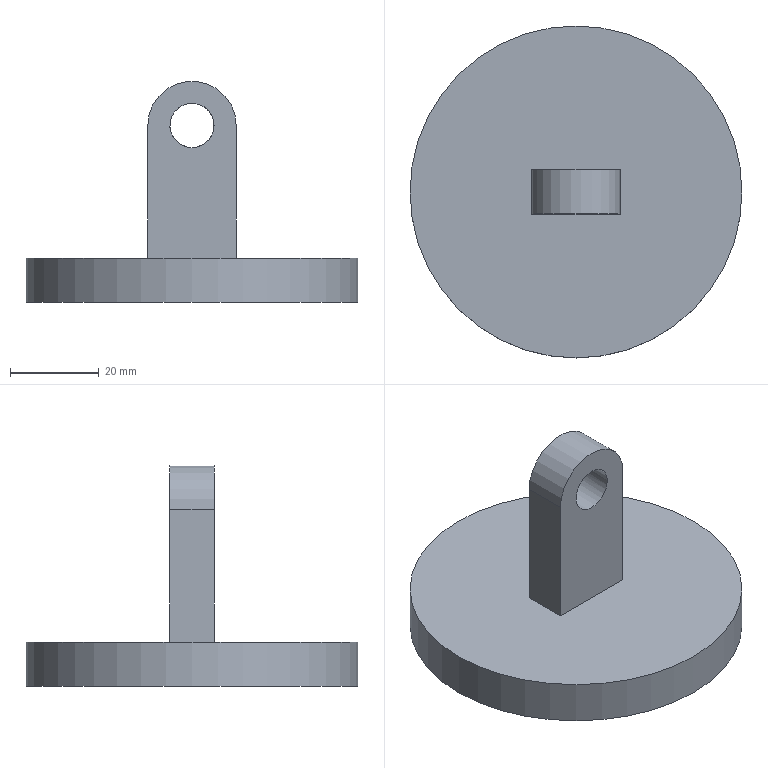Component | NX | CIRCLE_PISTON | 1 solid | 9 faces | box 75 x 75 x 50 mm | volume 50964 mm3 | plane 6 | cylinder 3 | commonest cylinder face diameters 75 x1 20 x1 10 x1
STEP:
#1=CARTESIAN_POINT('',(0.,0.,0.));
#2=DIRECTION('',(0.,0.,1.));
#3=DIRECTION('',(1.,0.,0.));
#4=AXIS2_PLACEMENT_3D('',#1,#2,#3);
#5=CARTESIAN_POINT('',(-162.5,20.,60.412));
#6=VERTEX_POINT('',#5);
#7=CARTESIAN_POINT('',(-200.,20.,60.412));
#8=DIRECTION('',(0.,0.,1.));
#9=DIRECTION('',(1.,0.,0.));
#10=AXIS2_PLACEMENT_3D('',#7,#8,#9);
#11=CIRCLE('',#10,37.5);
#12=CARTESIAN_POINT('',(-200.,20.,60.412));
#13=DIRECTION('',(0.,0.,1.));
#14=DIRECTION('',(1.,0.,0.));
#15=AXIS2_PLACEMENT_3D('',#12,#13,#14);
#16=PLANE('',#15);
#17=CARTESIAN_POINT('',(0.,0.));
#18=DIRECTION('',(1.,0.));
#19=AXIS2_PLACEMENT_2D('',#17,#18);
#20=CIRCLE('',#19,37.5);
#21=(GEOMETRIC_REPRESENTATION_CONTEXT(2)PARAMETRIC_REPRESENTATION_CONTEXT()REPRESENTATION_CONTEXT('',''));
#22=DEFINITIONAL_REPRESENTATION('',(#20),#21);
#23=PCURVE('',#16,#22);
#24=CARTESIAN_POINT('',(-200.,20.,60.412));
#25=DIRECTION('',(0.,0.,-1.));
#26=DIRECTION('',(-1.,0.,0.));
#27=AXIS2_PLACEMENT_3D('',#24,#25,#26);
#28=CYLINDRICAL_SURFACE('',#27,37.5);
#29=CARTESIAN_POINT('',(9.425,0.));
#30=DIRECTION('',(-1.,0.));
#31=VECTOR('',#30,1.);
#32=LINE('',#29,#31);
#33=(GEOMETRIC_REPRESENTATION_CONTEXT(2)PARAMETRIC_REPRESENTATION_CONTEXT()REPRESENTATION_CONTEXT('',''));
#34=DEFINITIONAL_REPRESENTATION('',(#32),#33);
#35=PCURVE('',#28,#34);
#36=SURFACE_CURVE('',#11,(#23,#35),.PCURVE_S1.);
#37=EDGE_CURVE('',#6,#6,#36,.T.);
#38=ORIENTED_EDGE('',*,*,#37,.T.);
#39=EDGE_LOOP('',(#38));
#40=FACE_BOUND('',#39,.T.);
#41=CARTESIAN_POINT('',(-210.,15.,60.412));
#42=VERTEX_POINT('',#41);
#43=CARTESIAN_POINT('',(-210.,25.,60.412));
#44=VERTEX_POINT('',#43);
#45=CARTESIAN_POINT('',(-210.,15.,60.412));
#46=DIRECTION('',(0.,1.,0.));
#47=VECTOR('',#46,1.);
#48=LINE('',#45,#47);
#49=CARTESIAN_POINT('',(-10.,-5.));
#50=DIRECTION('',(0.,1.));
#51=VECTOR('',#50,1.);
#52=LINE('',#49,#51);
#53=(GEOMETRIC_REPRESENTATION_CONTEXT(2)PARAMETRIC_REPRESENTATION_CONTEXT()REPRESENTATION_CONTEXT('',''));
#54=DEFINITIONAL_REPRESENTATION('',(#52),#53);
#55=PCURVE('',#16,#54);
#56=CARTESIAN_POINT('',(-210.,15.,90.412));
#57=DIRECTION('',(1.,0.,0.));
#58=DIRECTION('',(0.,0.,-1.));
#59=AXIS2_PLACEMENT_3D('',#56,#57,#58);
#60=PLANE('',#59);
#61=CARTESIAN_POINT('',(30.,0.));
#62=DIRECTION('',(0.,1.));
#63=VECTOR('',#62,1.);
#64=LINE('',#61,#63);
#65=(GEOMETRIC_REPRESENTATION_CONTEXT(2)PARAMETRIC_REPRESENTATION_CONTEXT()REPRESENTATION_CONTEXT('',''));
#66=DEFINITIONAL_REPRESENTATION('',(#64),#65);
#67=PCURVE('',#60,#66);
#68=SURFACE_CURVE('',#48,(#55,#67),.PCURVE_S1.);
#69=EDGE_CURVE('',#42,#44,#68,.T.);
#70=ORIENTED_EDGE('',*,*,#69,.T.);
#71=CARTESIAN_POINT('',(-190.,25.,60.412));
#72=VERTEX_POINT('',#71);
#73=CARTESIAN_POINT('',(-210.,25.,60.412));
#74=DIRECTION('',(1.,0.,-0.));
#75=VECTOR('',#74,1.);
#76=LINE('',#73,#75);
#77=CARTESIAN_POINT('',(-10.,5.));
#78=DIRECTION('',(1.,0.));
#79=VECTOR('',#78,1.);
#80=LINE('',#77,#79);
#81=(GEOMETRIC_REPRESENTATION_CONTEXT(2)PARAMETRIC_REPRESENTATION_CONTEXT()REPRESENTATION_CONTEXT('',''));
#82=DEFINITIONAL_REPRESENTATION('',(#80),#81);
#83=PCURVE('',#16,#82);
#84=CARTESIAN_POINT('',(-200.,25.,90.412));
#85=DIRECTION('',(0.,-1.,0.));
#86=DIRECTION('',(0.,0.,-1.));
#87=AXIS2_PLACEMENT_3D('',#84,#85,#86);
#88=PLANE('',#87);
#89=CARTESIAN_POINT('',(30.,-10.));
#90=DIRECTION('',(0.,1.));
#91=VECTOR('',#90,1.);
#92=LINE('',#89,#91);
#93=(GEOMETRIC_REPRESENTATION_CONTEXT(2)PARAMETRIC_REPRESENTATION_CONTEXT()REPRESENTATION_CONTEXT('',''));
#94=DEFINITIONAL_REPRESENTATION('',(#92),#93);
#95=PCURVE('',#88,#94);
#96=SURFACE_CURVE('',#76,(#83,#95),.PCURVE_S1.);
#97=EDGE_CURVE('',#44,#72,#96,.T.);
#98=ORIENTED_EDGE('',*,*,#97,.T.);
#99=CARTESIAN_POINT('',(-190.,15.,60.412));
#100=VERTEX_POINT('',#99);
#101=CARTESIAN_POINT('',(-190.,15.,60.412));
#102=DIRECTION('',(0.,1.,0.));
#103=VECTOR('',#102,1.);
#104=LINE('',#101,#103);
#105=CARTESIAN_POINT('',(10.,-5.));
#106=DIRECTION('',(0.,1.));
#107=VECTOR('',#106,1.);
#108=LINE('',#105,#107);
#109=(GEOMETRIC_REPRESENTATION_CONTEXT(2)PARAMETRIC_REPRESENTATION_CONTEXT()REPRESENTATION_CONTEXT('',''));
#110=DEFINITIONAL_REPRESENTATION('',(#108),#109);
#111=PCURVE('',#16,#110);
#112=CARTESIAN_POINT('',(-190.,15.,60.412));
#113=DIRECTION('',(-1.,0.,-0.));
#114=DIRECTION('',(-0.,0.,1.));
#115=AXIS2_PLACEMENT_3D('',#112,#113,#114);
#116=PLANE('',#115);
#117=CARTESIAN_POINT('',(0.,0.));
#118=DIRECTION('',(0.,1.));
#119=VECTOR('',#118,1.);
#120=LINE('',#117,#119);
#121=(GEOMETRIC_REPRESENTATION_CONTEXT(2)PARAMETRIC_REPRESENTATION_CONTEXT()REPRESENTATION_CONTEXT('',''));
#122=DEFINITIONAL_REPRESENTATION('',(#120),#121);
#123=PCURVE('',#116,#122);
#124=SURFACE_CURVE('',#104,(#111,#123),.PCURVE_S1.);
#125=EDGE_CURVE('',#100,#72,#124,.T.);
#126=ORIENTED_EDGE('',*,*,#125,.F.);
#127=CARTESIAN_POINT('',(-210.,15.,60.412));
#128=DIRECTION('',(1.,0.,-0.));
#129=VECTOR('',#128,1.);
#130=LINE('',#127,#129);
#131=CARTESIAN_POINT('',(-10.,-5.));
#132=DIRECTION('',(1.,0.));
#133=VECTOR('',#132,1.);
#134=LINE('',#131,#133);
#135=(GEOMETRIC_REPRESENTATION_CONTEXT(2)PARAMETRIC_REPRESENTATION_CONTEXT()REPRESENTATION_CONTEXT('',''));
#136=DEFINITIONAL_REPRESENTATION('',(#134),#135);
#137=PCURVE('',#16,#136);
#138=CARTESIAN_POINT('',(-200.,15.,90.412));
#139=DIRECTION('',(0.,-1.,0.));
#140=DIRECTION('',(0.,0.,-1.));
#141=AXIS2_PLACEMENT_3D('',#138,#139,#140);
#142=PLANE('',#141);
#143=CARTESIAN_POINT('',(30.,-10.));
#144=DIRECTION('',(0.,1.));
#145=VECTOR('',#144,1.);
#146=LINE('',#143,#145);
#147=(GEOMETRIC_REPRESENTATION_CONTEXT(2)PARAMETRIC_REPRESENTATION_CONTEXT()REPRESENTATION_CONTEXT('',''));
#148=DEFINITIONAL_REPRESENTATION('',(#146),#147);
#149=PCURVE('',#142,#148);
#150=SURFACE_CURVE('',#130,(#137,#149),.PCURVE_S1.);
#151=EDGE_CURVE('',#42,#100,#150,.T.);
#152=ORIENTED_EDGE('',*,*,#151,.F.);
#153=EDGE_LOOP('',(#70,#98,#126,#152));
#154=FACE_BOUND('',#153,.T.);
#155=ADVANCED_FACE('',(#40,#154),#16,.T.);
#156=ORIENTED_EDGE('',*,*,#37,.F.);
#157=CARTESIAN_POINT('',(-162.5,20.,50.412));
#158=VERTEX_POINT('',#157);
#159=CARTESIAN_POINT('',(-162.5,20.,60.412));
#160=CARTESIAN_POINT('',(-162.5,20.,50.412));
#161=B_SPLINE_CURVE_WITH_KNOTS('',1,(#159,#160),.UNSPECIFIED.,.F.,.F.,(2,2),(0.,10.),.PIECEWISE_BEZIER_KNOTS.);
#162=CARTESIAN_POINT('',(9.425,0.));
#163=DIRECTION('',(0.,1.));
#164=VECTOR('',#163,1.);
#165=LINE('',#162,#164);
#166=(GEOMETRIC_REPRESENTATION_CONTEXT(2)PARAMETRIC_REPRESENTATION_CONTEXT()REPRESENTATION_CONTEXT('',''));
#167=DEFINITIONAL_REPRESENTATION('',(#165),#166);
#168=PCURVE('',#28,#167);
#169=CARTESIAN_POINT('',(3.142,0.));
#170=DIRECTION('',(0.,1.));
#171=VECTOR('',#170,1.);
#172=LINE('',#169,#171);
#173=(GEOMETRIC_REPRESENTATION_CONTEXT(2)PARAMETRIC_REPRESENTATION_CONTEXT()REPRESENTATION_CONTEXT('',''));
#174=DEFINITIONAL_REPRESENTATION('',(#172),#173);
#175=PCURVE('',#28,#174);
#176=SEAM_CURVE('',#161,(#168,#175),.PCURVE_S1.);
#177=EDGE_CURVE('',#6,#158,#176,.T.);
#178=ORIENTED_EDGE('',*,*,#177,.T.);
#179=CARTESIAN_POINT('',(-200.,20.,50.412));
#180=DIRECTION('',(0.,0.,1.));
#181=DIRECTION('',(1.,0.,0.));
#182=AXIS2_PLACEMENT_3D('',#179,#180,#181);
#183=CIRCLE('',#182,37.5);
#184=CARTESIAN_POINT('',(9.425,10.));
#185=DIRECTION('',(-1.,0.));
#186=VECTOR('',#185,1.);
#187=LINE('',#184,#186);
#188=(GEOMETRIC_REPRESENTATION_CONTEXT(2)PARAMETRIC_REPRESENTATION_CONTEXT()REPRESENTATION_CONTEXT('',''));
#189=DEFINITIONAL_REPRESENTATION('',(#187),#188);
#190=PCURVE('',#28,#189);
#191=CARTESIAN_POINT('',(-200.,20.,50.412));
#192=DIRECTION('',(0.,0.,1.));
#193=DIRECTION('',(1.,0.,0.));
#194=AXIS2_PLACEMENT_3D('',#191,#192,#193);
#195=PLANE('',#194);
#196=CARTESIAN_POINT('',(0.,0.));
#197=DIRECTION('',(1.,0.));
#198=AXIS2_PLACEMENT_2D('',#196,#197);
#199=CIRCLE('',#198,37.5);
#200=(GEOMETRIC_REPRESENTATION_CONTEXT(2)PARAMETRIC_REPRESENTATION_CONTEXT()REPRESENTATION_CONTEXT('',''));
#201=DEFINITIONAL_REPRESENTATION('',(#199),#200);
#202=PCURVE('',#195,#201);
#203=SURFACE_CURVE('',#183,(#190,#202),.PCURVE_S1.);
#204=EDGE_CURVE('',#158,#158,#203,.T.);
#205=ORIENTED_EDGE('',*,*,#204,.T.);
#206=ORIENTED_EDGE('',*,*,#177,.F.);
#207=EDGE_LOOP('',(#156,#178,#205,#206));
#208=FACE_BOUND('',#207,.T.);
#209=ADVANCED_FACE('',(#208),#28,.T.);
#210=ORIENTED_EDGE('',*,*,#204,.F.);
#211=EDGE_LOOP('',(#210));
#212=FACE_BOUND('',#211,.T.);
#213=ADVANCED_FACE('',(#212),#195,.F.);
#214=CARTESIAN_POINT('',(-210.,25.,90.412));
#215=VERTEX_POINT('',#214);
#216=CARTESIAN_POINT('',(-210.,25.,90.412));
#217=DIRECTION('',(0.,0.,-1.));
#218=VECTOR('',#217,1.);
#219=LINE('',#216,#218);
#220=CARTESIAN_POINT('',(0.,10.));
#221=DIRECTION('',(1.,0.));
#222=VECTOR('',#221,1.);
#223=LINE('',#220,#222);
#224=(GEOMETRIC_REPRESENTATION_CONTEXT(2)PARAMETRIC_REPRESENTATION_CONTEXT()REPRESENTATION_CONTEXT('',''));
#225=DEFINITIONAL_REPRESENTATION('',(#223),#224);
#226=PCURVE('',#60,#225);
#227=CARTESIAN_POINT('',(0.,-10.));
#228=DIRECTION('',(1.,0.));
#229=VECTOR('',#228,1.);
#230=LINE('',#227,#229);
#231=(GEOMETRIC_REPRESENTATION_CONTEXT(2)PARAMETRIC_REPRESENTATION_CONTEXT()REPRESENTATION_CONTEXT('',''));
#232=DEFINITIONAL_REPRESENTATION('',(#230),#231);
#233=PCURVE('',#88,#232);
#234=SURFACE_CURVE('',#219,(#226,#233),.PCURVE_S1.);
#235=EDGE_CURVE('',#215,#44,#234,.T.);
#236=ORIENTED_EDGE('',*,*,#235,.T.);
#237=ORIENTED_EDGE('',*,*,#69,.F.);
#238=CARTESIAN_POINT('',(-210.,15.,90.412));
#239=VERTEX_POINT('',#238);
#240=CARTESIAN_POINT('',(-210.,15.,90.412));
#241=DIRECTION('',(0.,0.,-1.));
#242=VECTOR('',#241,1.);
#243=LINE('',#240,#242);
#244=CARTESIAN_POINT('',(0.,0.));
#245=DIRECTION('',(1.,0.));
#246=VECTOR('',#245,1.);
#247=LINE('',#244,#246);
#248=(GEOMETRIC_REPRESENTATION_CONTEXT(2)PARAMETRIC_REPRESENTATION_CONTEXT()REPRESENTATION_CONTEXT('',''));
#249=DEFINITIONAL_REPRESENTATION('',(#247),#248);
#250=PCURVE('',#60,#249);
#251=CARTESIAN_POINT('',(0.,-10.));
#252=DIRECTION('',(1.,0.));
#253=VECTOR('',#252,1.);
#254=LINE('',#251,#253);
#255=(GEOMETRIC_REPRESENTATION_CONTEXT(2)PARAMETRIC_REPRESENTATION_CONTEXT()REPRESENTATION_CONTEXT('',''));
#256=DEFINITIONAL_REPRESENTATION('',(#254),#255);
#257=PCURVE('',#142,#256);
#258=SURFACE_CURVE('',#243,(#250,#257),.PCURVE_S1.);
#259=EDGE_CURVE('',#239,#42,#258,.T.);
#260=ORIENTED_EDGE('',*,*,#259,.F.);
#261=CARTESIAN_POINT('',(-210.,15.,90.412));
#262=DIRECTION('',(0.,1.,0.));
#263=VECTOR('',#262,1.);
#264=LINE('',#261,#263);
#265=CARTESIAN_POINT('',(0.,0.));
#266=DIRECTION('',(0.,1.));
#267=VECTOR('',#266,1.);
#268=LINE('',#265,#267);
#269=(GEOMETRIC_REPRESENTATION_CONTEXT(2)PARAMETRIC_REPRESENTATION_CONTEXT()REPRESENTATION_CONTEXT('',''));
#270=DEFINITIONAL_REPRESENTATION('',(#268),#269);
#271=PCURVE('',#60,#270);
#272=CARTESIAN_POINT('',(-200.,15.,90.412));
#273=DIRECTION('',(0.,1.,0.));
#274=DIRECTION('',(0.,0.,1.));
#275=AXIS2_PLACEMENT_3D('',#272,#273,#274);
#276=CYLINDRICAL_SURFACE('',#275,10.);
#277=CARTESIAN_POINT('',(-1.571,0.));
#278=DIRECTION('',(0.,1.));
#279=VECTOR('',#278,1.);
#280=LINE('',#277,#279);
#281=(GEOMETRIC_REPRESENTATION_CONTEXT(2)PARAMETRIC_REPRESENTATION_CONTEXT()REPRESENTATION_CONTEXT('',''));
#282=DEFINITIONAL_REPRESENTATION('',(#280),#281);
#283=PCURVE('',#276,#282);
#284=SURFACE_CURVE('',#264,(#271,#283),.PCURVE_S1.);
#285=EDGE_CURVE('',#239,#215,#284,.T.);
#286=ORIENTED_EDGE('',*,*,#285,.T.);
#287=EDGE_LOOP('',(#236,#237,#260,#286));
#288=FACE_BOUND('',#287,.T.);
#289=ADVANCED_FACE('',(#288),#60,.F.);
#290=CARTESIAN_POINT('',(-190.,25.,90.412));
#291=VERTEX_POINT('',#290);
#292=CARTESIAN_POINT('',(-190.,25.,60.412));
#293=DIRECTION('',(-0.,0.,1.));
#294=VECTOR('',#293,1.);
#295=LINE('',#292,#294);
#296=CARTESIAN_POINT('',(0.,10.));
#297=DIRECTION('',(1.,0.));
#298=VECTOR('',#297,1.);
#299=LINE('',#296,#298);
#300=(GEOMETRIC_REPRESENTATION_CONTEXT(2)PARAMETRIC_REPRESENTATION_CONTEXT()REPRESENTATION_CONTEXT('',''));
#301=DEFINITIONAL_REPRESENTATION('',(#299),#300);
#302=PCURVE('',#116,#301);
#303=CARTESIAN_POINT('',(30.,10.));
#304=DIRECTION('',(-1.,-0.));
#305=VECTOR('',#304,1.);
#306=LINE('',#303,#305);
#307=(GEOMETRIC_REPRESENTATION_CONTEXT(2)PARAMETRIC_REPRESENTATION_CONTEXT()REPRESENTATION_CONTEXT('',''));
#308=DEFINITIONAL_REPRESENTATION('',(#306),#307);
#309=PCURVE('',#88,#308);
#310=SURFACE_CURVE('',#295,(#302,#309),.PCURVE_S1.);
#311=EDGE_CURVE('',#72,#291,#310,.T.);
#312=ORIENTED_EDGE('',*,*,#311,.T.);
#313=CARTESIAN_POINT('',(-190.,15.,90.412));
#314=VERTEX_POINT('',#313);
#315=CARTESIAN_POINT('',(-190.,15.,90.412));
#316=DIRECTION('',(0.,1.,0.));
#317=VECTOR('',#316,1.);
#318=LINE('',#315,#317);
#319=CARTESIAN_POINT('',(30.,0.));
#320=DIRECTION('',(0.,1.));
#321=VECTOR('',#320,1.);
#322=LINE('',#319,#321);
#323=(GEOMETRIC_REPRESENTATION_CONTEXT(2)PARAMETRIC_REPRESENTATION_CONTEXT()REPRESENTATION_CONTEXT('',''));
#324=DEFINITIONAL_REPRESENTATION('',(#322),#323);
#325=PCURVE('',#116,#324);
#326=CARTESIAN_POINT('',(1.571,0.));
#327=DIRECTION('',(0.,1.));
#328=VECTOR('',#327,1.);
#329=LINE('',#326,#328);
#330=(GEOMETRIC_REPRESENTATION_CONTEXT(2)PARAMETRIC_REPRESENTATION_CONTEXT()REPRESENTATION_CONTEXT('',''));
#331=DEFINITIONAL_REPRESENTATION('',(#329),#330);
#332=PCURVE('',#276,#331);
#333=SURFACE_CURVE('',#318,(#325,#332),.PCURVE_S1.);
#334=EDGE_CURVE('',#314,#291,#333,.T.);
#335=ORIENTED_EDGE('',*,*,#334,.F.);
#336=CARTESIAN_POINT('',(-190.,15.,60.412));
#337=DIRECTION('',(-0.,0.,1.));
#338=VECTOR('',#337,1.);
#339=LINE('',#336,#338);
#340=CARTESIAN_POINT('',(0.,0.));
#341=DIRECTION('',(1.,0.));
#342=VECTOR('',#341,1.);
#343=LINE('',#340,#342);
#344=(GEOMETRIC_REPRESENTATION_CONTEXT(2)PARAMETRIC_REPRESENTATION_CONTEXT()REPRESENTATION_CONTEXT('',''));
#345=DEFINITIONAL_REPRESENTATION('',(#343),#344);
#346=PCURVE('',#116,#345);
#347=CARTESIAN_POINT('',(30.,10.));
#348=DIRECTION('',(-1.,-0.));
#349=VECTOR('',#348,1.);
#350=LINE('',#347,#349);
#351=(GEOMETRIC_REPRESENTATION_CONTEXT(2)PARAMETRIC_REPRESENTATION_CONTEXT()REPRESENTATION_CONTEXT('',''));
#352=DEFINITIONAL_REPRESENTATION('',(#350),#351);
#353=PCURVE('',#142,#352);
#354=SURFACE_CURVE('',#339,(#346,#353),.PCURVE_S1.);
#355=EDGE_CURVE('',#100,#314,#354,.T.);
#356=ORIENTED_EDGE('',*,*,#355,.F.);
#357=ORIENTED_EDGE('',*,*,#125,.T.);
#358=EDGE_LOOP('',(#312,#335,#356,#357));
#359=FACE_BOUND('',#358,.T.);
#360=ADVANCED_FACE('',(#359),#116,.F.);
#361=CARTESIAN_POINT('',(-200.,25.,90.412));
#362=DIRECTION('',(0.,-1.,0.));
#363=DIRECTION('',(1.,0.,0.));
#364=AXIS2_PLACEMENT_3D('',#361,#362,#363);
#365=CIRCLE('',#364,10.);
#366=CARTESIAN_POINT('',(1.571,10.));
#367=DIRECTION('',(-1.,0.));
#368=VECTOR('',#367,1.);
#369=LINE('',#366,#368);
#370=(GEOMETRIC_REPRESENTATION_CONTEXT(2)PARAMETRIC_REPRESENTATION_CONTEXT()REPRESENTATION_CONTEXT('',''));
#371=DEFINITIONAL_REPRESENTATION('',(#369),#370);
#372=PCURVE('',#276,#371);
#373=CARTESIAN_POINT('',(0.,0.));
#374=DIRECTION('',(0.,1.));
#375=AXIS2_PLACEMENT_2D('',#373,#374);
#376=CIRCLE('',#375,10.);
#377=(GEOMETRIC_REPRESENTATION_CONTEXT(2)PARAMETRIC_REPRESENTATION_CONTEXT()REPRESENTATION_CONTEXT('',''));
#378=DEFINITIONAL_REPRESENTATION('',(#376),#377);
#379=PCURVE('',#88,#378);
#380=SURFACE_CURVE('',#365,(#372,#379),.PCURVE_S1.);
#381=EDGE_CURVE('',#291,#215,#380,.T.);
#382=ORIENTED_EDGE('',*,*,#381,.T.);
#383=ORIENTED_EDGE('',*,*,#285,.F.);
#384=CARTESIAN_POINT('',(-200.,15.,90.412));
#385=DIRECTION('',(0.,-1.,0.));
#386=DIRECTION('',(1.,0.,0.));
#387=AXIS2_PLACEMENT_3D('',#384,#385,#386);
#388=CIRCLE('',#387,10.);
#389=CARTESIAN_POINT('',(1.571,0.));
#390=DIRECTION('',(-1.,0.));
#391=VECTOR('',#390,1.);
#392=LINE('',#389,#391);
#393=(GEOMETRIC_REPRESENTATION_CONTEXT(2)PARAMETRIC_REPRESENTATION_CONTEXT()REPRESENTATION_CONTEXT('',''));
#394=DEFINITIONAL_REPRESENTATION('',(#392),#393);
#395=PCURVE('',#276,#394);
#396=CARTESIAN_POINT('',(0.,0.));
#397=DIRECTION('',(0.,1.));
#398=AXIS2_PLACEMENT_2D('',#396,#397);
#399=CIRCLE('',#398,10.);
#400=(GEOMETRIC_REPRESENTATION_CONTEXT(2)PARAMETRIC_REPRESENTATION_CONTEXT()REPRESENTATION_CONTEXT('',''));
#401=DEFINITIONAL_REPRESENTATION('',(#399),#400);
#402=PCURVE('',#142,#401);
#403=SURFACE_CURVE('',#388,(#395,#402),.PCURVE_S1.);
#404=EDGE_CURVE('',#314,#239,#403,.T.);
#405=ORIENTED_EDGE('',*,*,#404,.F.);
#406=ORIENTED_EDGE('',*,*,#334,.T.);
#407=EDGE_LOOP('',(#382,#383,#405,#406));
#408=FACE_BOUND('',#407,.T.);
#409=ADVANCED_FACE('',(#408),#276,.T.);
#410=CARTESIAN_POINT('',(-195.,15.,90.412));
#411=VERTEX_POINT('',#410);
#412=CARTESIAN_POINT('',(-200.,15.,85.412));
#413=VERTEX_POINT('',#412);
#414=CARTESIAN_POINT('',(-200.,15.,90.412));
#415=DIRECTION('',(0.,-1.,0.));
#416=DIRECTION('',(1.,0.,0.));
#417=AXIS2_PLACEMENT_3D('',#414,#415,#416);
#418=CIRCLE('',#417,5.);
#419=CARTESIAN_POINT('',(0.,0.));
#420=DIRECTION('',(0.,1.));
#421=AXIS2_PLACEMENT_2D('',#419,#420);
#422=CIRCLE('',#421,5.);
#423=(GEOMETRIC_REPRESENTATION_CONTEXT(2)PARAMETRIC_REPRESENTATION_CONTEXT()REPRESENTATION_CONTEXT('',''));
#424=DEFINITIONAL_REPRESENTATION('',(#422),#423);
#425=PCURVE('',#142,#424);
#426=CARTESIAN_POINT('',(-200.,114.,90.412));
#427=DIRECTION('',(0.,-1.,0.));
#428=DIRECTION('',(0.,0.,-1.));
#429=AXIS2_PLACEMENT_3D('',#426,#427,#428);
#430=CYLINDRICAL_SURFACE('',#429,5.);
#431=CARTESIAN_POINT('',(1.571,99.));
#432=DIRECTION('',(1.,0.));
#433=VECTOR('',#432,1.);
#434=LINE('',#431,#433);
#435=(GEOMETRIC_REPRESENTATION_CONTEXT(2)PARAMETRIC_REPRESENTATION_CONTEXT()REPRESENTATION_CONTEXT('',''));
#436=DEFINITIONAL_REPRESENTATION('',(#434),#435);
#437=PCURVE('',#430,#436);
#438=SURFACE_CURVE('',#418,(#425,#437),.PCURVE_S1.);
#439=EDGE_CURVE('',#411,#413,#438,.T.);
#440=ORIENTED_EDGE('',*,*,#439,.F.);
#441=CARTESIAN_POINT('',(-200.,15.,90.412));
#442=DIRECTION('',(0.,-1.,0.));
#443=DIRECTION('',(1.,0.,0.));
#444=AXIS2_PLACEMENT_3D('',#441,#442,#443);
#445=CIRCLE('',#444,5.);
#446=CARTESIAN_POINT('',(0.,0.));
#447=DIRECTION('',(0.,1.));
#448=AXIS2_PLACEMENT_2D('',#446,#447);
#449=CIRCLE('',#448,5.);
#450=(GEOMETRIC_REPRESENTATION_CONTEXT(2)PARAMETRIC_REPRESENTATION_CONTEXT()REPRESENTATION_CONTEXT('',''));
#451=DEFINITIONAL_REPRESENTATION('',(#449),#450);
#452=PCURVE('',#142,#451);
#453=CARTESIAN_POINT('',(-4.712,99.));
#454=DIRECTION('',(1.,0.));
#455=VECTOR('',#454,1.);
#456=LINE('',#453,#455);
#457=(GEOMETRIC_REPRESENTATION_CONTEXT(2)PARAMETRIC_REPRESENTATION_CONTEXT()REPRESENTATION_CONTEXT('',''));
#458=DEFINITIONAL_REPRESENTATION('',(#456),#457);
#459=PCURVE('',#430,#458);
#460=SURFACE_CURVE('',#445,(#452,#459),.PCURVE_S1.);
#461=EDGE_CURVE('',#413,#411,#460,.T.);
#462=ORIENTED_EDGE('',*,*,#461,.F.);
#463=EDGE_LOOP('',(#440,#462));
#464=FACE_BOUND('',#463,.T.);
#465=ORIENTED_EDGE('',*,*,#259,.T.);
#466=ORIENTED_EDGE('',*,*,#151,.T.);
#467=ORIENTED_EDGE('',*,*,#355,.T.);
#468=ORIENTED_EDGE('',*,*,#404,.T.);
#469=EDGE_LOOP('',(#465,#466,#467,#468));
#470=FACE_BOUND('',#469,.T.);
#471=ADVANCED_FACE('',(#464,#470),#142,.T.);
#472=CARTESIAN_POINT('',(-200.,25.,85.412));
#473=VERTEX_POINT('',#472);
#474=CARTESIAN_POINT('',(-200.,25.,90.412));
#475=DIRECTION('',(0.,1.,0.));
#476=DIRECTION('',(0.,0.,-1.));
#477=AXIS2_PLACEMENT_3D('',#474,#475,#476);
#478=CIRCLE('',#477,5.);
#479=CARTESIAN_POINT('',(5.,0.));
#480=CARTESIAN_POINT('',(5.,-8.66));
#481=CARTESIAN_POINT('',(-2.5,-4.33));
#482=CARTESIAN_POINT('',(-10.,-0.));
#483=CARTESIAN_POINT('',(-2.5,4.33));
#484=CARTESIAN_POINT('',(5.,8.66));
#485=CARTESIAN_POINT('',(5.,0.));
#486=(BOUNDED_CURVE()B_SPLINE_CURVE(2,(#479,#480,#481,#482,#483,#484,#485),.UNSPECIFIED.,.T.,.F.)B_SPLINE_CURVE_WITH_KNOTS((1,2,2,2,2,1),(-2.094,0.,2.094,4.189,6.283,8.378),.UNSPECIFIED.)CURVE()GEOMETRIC_REPRESENTATION_ITEM()RATIONAL_B_SPLINE_CURVE((1.,0.5,1.,0.5,1.,0.5,1.))REPRESENTATION_ITEM(''));
#487=(GEOMETRIC_REPRESENTATION_CONTEXT(2)PARAMETRIC_REPRESENTATION_CONTEXT()REPRESENTATION_CONTEXT('',''));
#488=DEFINITIONAL_REPRESENTATION('',(#486),#487);
#489=PCURVE('',#88,#488);
#490=CARTESIAN_POINT('',(6.283,89.));
#491=DIRECTION('',(-1.,0.));
#492=VECTOR('',#491,1.);
#493=LINE('',#490,#492);
#494=(GEOMETRIC_REPRESENTATION_CONTEXT(2)PARAMETRIC_REPRESENTATION_CONTEXT()REPRESENTATION_CONTEXT('',''));
#495=DEFINITIONAL_REPRESENTATION('',(#493),#494);
#496=PCURVE('',#430,#495);
#497=SURFACE_CURVE('',#478,(#489,#496),.PCURVE_S1.);
#498=EDGE_CURVE('',#473,#473,#497,.T.);
#499=ORIENTED_EDGE('',*,*,#498,.F.);
#500=EDGE_LOOP('',(#499));
#501=FACE_BOUND('',#500,.T.);
#502=ORIENTED_EDGE('',*,*,#235,.F.);
#503=ORIENTED_EDGE('',*,*,#381,.F.);
#504=ORIENTED_EDGE('',*,*,#311,.F.);
#505=ORIENTED_EDGE('',*,*,#97,.F.);
#506=EDGE_LOOP('',(#502,#503,#504,#505));
#507=FACE_BOUND('',#506,.T.);
#508=ADVANCED_FACE('',(#501,#507),#88,.F.);
#509=ORIENTED_EDGE('',*,*,#498,.F.);
#510=CARTESIAN_POINT('',(-200.,25.,85.412));
#511=CARTESIAN_POINT('',(-200.,15.,85.412));
#512=B_SPLINE_CURVE_WITH_KNOTS('',1,(#510,#511),.UNSPECIFIED.,.F.,.F.,(2,2),(89.,99.),.PIECEWISE_BEZIER_KNOTS.);
#513=CARTESIAN_POINT('',(6.283,0.));
#514=DIRECTION('',(0.,1.));
#515=VECTOR('',#514,1.);
#516=LINE('',#513,#515);
#517=(GEOMETRIC_REPRESENTATION_CONTEXT(2)PARAMETRIC_REPRESENTATION_CONTEXT()REPRESENTATION_CONTEXT('',''));
#518=DEFINITIONAL_REPRESENTATION('',(#516),#517);
#519=PCURVE('',#430,#518);
#520=CARTESIAN_POINT('',(0.,0.));
#521=DIRECTION('',(0.,1.));
#522=VECTOR('',#521,1.);
#523=LINE('',#520,#522);
#524=(GEOMETRIC_REPRESENTATION_CONTEXT(2)PARAMETRIC_REPRESENTATION_CONTEXT()REPRESENTATION_CONTEXT('',''));
#525=DEFINITIONAL_REPRESENTATION('',(#523),#524);
#526=PCURVE('',#430,#525);
#527=SEAM_CURVE('',#512,(#519,#526),.PCURVE_S1.);
#528=EDGE_CURVE('',#473,#413,#527,.T.);
#529=ORIENTED_EDGE('',*,*,#528,.T.);
#530=ORIENTED_EDGE('',*,*,#439,.F.);
#531=ORIENTED_EDGE('',*,*,#461,.F.);
#532=ORIENTED_EDGE('',*,*,#528,.F.);
#533=EDGE_LOOP('',(#509,#529,#530,#531,#532));
#534=FACE_BOUND('',#533,.F.);
#535=ADVANCED_FACE('',(#534),#430,.F.);
#536=CLOSED_SHELL('',(#155,#209,#213,#289,#360,#409,#471,#508,#535));
#537=MANIFOLD_SOLID_BREP('',#536);
#538=(LENGTH_UNIT()NAMED_UNIT(*)SI_UNIT(.MILLI.,.METRE.));
#539=UNCERTAINTY_MEASURE_WITH_UNIT(LENGTH_MEASURE(0.000002),#538,'','');
#540=(NAMED_UNIT(*)PLANE_ANGLE_UNIT()SI_UNIT($,.RADIAN.));
#541=(NAMED_UNIT(*)SI_UNIT($,.STERADIAN.)SOLID_ANGLE_UNIT());
#542=(GEOMETRIC_REPRESENTATION_CONTEXT(3)GLOBAL_UNCERTAINTY_ASSIGNED_CONTEXT((#539))GLOBAL_UNIT_ASSIGNED_CONTEXT((#538,#540,#541))REPRESENTATION_CONTEXT('',''));
#543=ADVANCED_BREP_SHAPE_REPRESENTATION('',(#4,#537),#542);